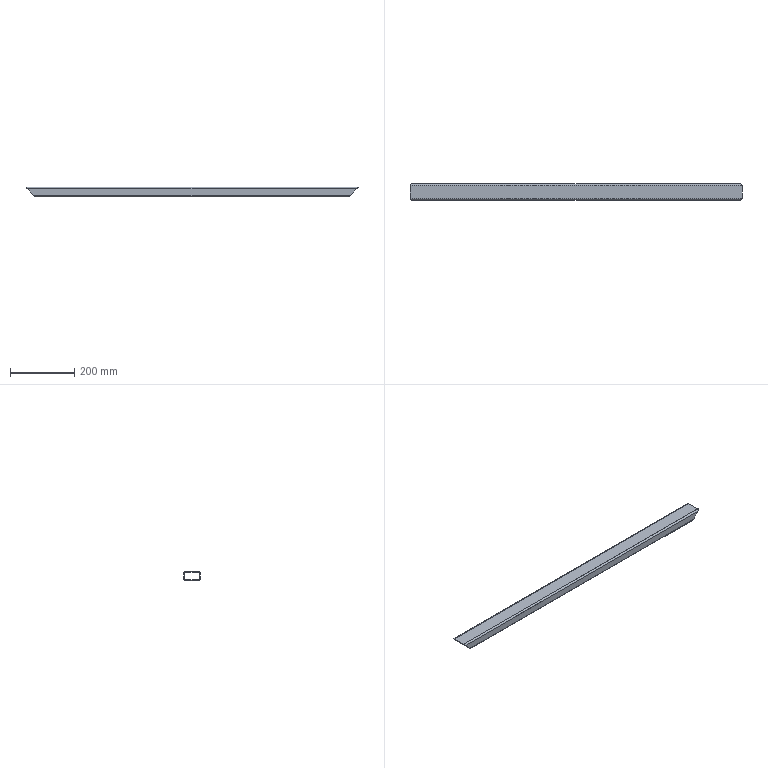Component | SolidWorks | Frame-1_SquareTube1-1 | 1 solid | 18 faces | box 1030 x 50 x 30 mm | volume 371551 mm3 | plane 10 | cylinder 8 | commonest cylinder face diameters 10.4 x4 5.2 x4
STEP:
#1=COLOUR_RGB('',0.7922,0.8196,0.9333);
#2=FILL_AREA_STYLE_COLOUR('',#1);
#3=FILL_AREA_STYLE('',(#2));
#4=SURFACE_STYLE_FILL_AREA(#3);
#5=SURFACE_SIDE_STYLE('',(#4));
#6=SURFACE_STYLE_USAGE(.BOTH.,#5);
#7=PRESENTATION_STYLE_ASSIGNMENT((#6));
#8=CARTESIAN_POINT('',(20.276,-0.7795,7.48));
#9=VERTEX_POINT('',#8);
#10=CARTESIAN_POINT('',(-20.276,-0.7795,7.48));
#11=VERTEX_POINT('',#10);
#12=CARTESIAN_POINT('',(19.685,-0.7795,7.48));
#13=DIRECTION('',(-1.,0.,0.));
#14=VECTOR('',#13,39.37);
#15=LINE('',#12,#14);
#16=EDGE_CURVE('',#9,#11,#15,.T.);
#17=ORIENTED_EDGE('',*,*,#16,.F.);
#18=CARTESIAN_POINT('',(20.276,0.7795,7.48));
#19=VERTEX_POINT('',#18);
#20=CARTESIAN_POINT('',(20.276,-0.7795,7.48));
#21=DIRECTION('',(0.,-1.,0.));
#22=VECTOR('',#21,39.37);
#23=LINE('',#20,#22);
#24=EDGE_CURVE('',#19,#9,#23,.T.);
#25=ORIENTED_EDGE('',*,*,#24,.F.);
#26=CARTESIAN_POINT('',(-20.276,0.7795,7.48));
#27=VERTEX_POINT('',#26);
#28=CARTESIAN_POINT('',(19.685,0.7795,7.48));
#29=DIRECTION('',(1.,0.,0.));
#30=VECTOR('',#29,39.37);
#31=LINE('',#28,#30);
#32=EDGE_CURVE('',#27,#19,#31,.T.);
#33=ORIENTED_EDGE('',*,*,#32,.F.);
#34=CARTESIAN_POINT('',(-20.276,-0.7795,7.48));
#35=DIRECTION('',(0.,1.,0.));
#36=VECTOR('',#35,39.37);
#37=LINE('',#34,#36);
#38=EDGE_CURVE('',#11,#27,#37,.T.);
#39=ORIENTED_EDGE('',*,*,#38,.F.);
#40=EDGE_LOOP('',(#17,#25,#33,#39));
#41=FACE_OUTER_BOUND('',#40,.T.);
#42=CARTESIAN_POINT('',(19.685,-0.7795,7.48));
#43=DIRECTION('',(0.,0.,-1.));
#44=DIRECTION('',(-1.,0.,0.));
#45=AXIS2_PLACEMENT_3D('',#42,#43,#44);
#46=PLANE('',#45);
#47=ADVANCED_FACE('',(#41),#46,.F.);
#48=ORIENTED_EDGE('',*,*,#38,.T.);
#49=CARTESIAN_POINT('',(-20.071,0.9843,7.276));
#50=VERTEX_POINT('',#49);
#51=CARTESIAN_POINT('',(-20.276,0.7795,7.48));
#52=CARTESIAN_POINT('',(-20.276,0.8995,7.48));
#53=CARTESIAN_POINT('',(-20.191,0.9843,7.396));
#54=CARTESIAN_POINT('',(-20.071,0.9843,7.276));
#55=(BOUNDED_CURVE()B_SPLINE_CURVE(3,(#51,#52,#53,#54),.UNSPECIFIED.,.F.,.F.)B_SPLINE_CURVE_WITH_KNOTS((4,4),(0.,1.571),.UNSPECIFIED.)CURVE()GEOMETRIC_REPRESENTATION_ITEM()RATIONAL_B_SPLINE_CURVE((1.,0.8047,0.8047,1.))REPRESENTATION_ITEM(''));
#56=EDGE_CURVE('',#27,#50,#55,.T.);
#57=ORIENTED_EDGE('',*,*,#56,.T.);
#58=CARTESIAN_POINT('',(-19.299,0.9843,6.504));
#59=VERTEX_POINT('',#58);
#60=CARTESIAN_POINT('',(-19.685,0.9843,6.89));
#61=DIRECTION('',(0.7071,0.,-0.7071));
#62=VECTOR('',#61,39.37);
#63=LINE('',#60,#62);
#64=EDGE_CURVE('',#50,#59,#63,.T.);
#65=ORIENTED_EDGE('',*,*,#64,.T.);
#66=CARTESIAN_POINT('',(-19.094,0.7795,6.299));
#67=VERTEX_POINT('',#66);
#68=CARTESIAN_POINT('',(-19.299,0.9843,6.504));
#69=CARTESIAN_POINT('',(-19.179,0.9843,6.384));
#70=CARTESIAN_POINT('',(-19.094,0.8995,6.299));
#71=CARTESIAN_POINT('',(-19.094,0.7795,6.299));
#72=(BOUNDED_CURVE()B_SPLINE_CURVE(3,(#68,#69,#70,#71),.UNSPECIFIED.,.F.,.T.)B_SPLINE_CURVE_WITH_KNOTS((4,4),(1.571,3.142),.UNSPECIFIED.)CURVE()GEOMETRIC_REPRESENTATION_ITEM()RATIONAL_B_SPLINE_CURVE((1.,0.8047,0.8047,1.))REPRESENTATION_ITEM(''));
#73=EDGE_CURVE('',#59,#67,#72,.T.);
#74=ORIENTED_EDGE('',*,*,#73,.T.);
#75=CARTESIAN_POINT('',(-19.094,-0.7795,6.299));
#76=VERTEX_POINT('',#75);
#77=CARTESIAN_POINT('',(-19.094,0.,6.299));
#78=DIRECTION('',(0.,-1.,0.));
#79=VECTOR('',#78,39.37);
#80=LINE('',#77,#79);
#81=EDGE_CURVE('',#67,#76,#80,.T.);
#82=ORIENTED_EDGE('',*,*,#81,.T.);
#83=CARTESIAN_POINT('',(-19.299,-0.9843,6.504));
#84=VERTEX_POINT('',#83);
#85=CARTESIAN_POINT('',(-19.094,-0.7795,6.299));
#86=CARTESIAN_POINT('',(-19.094,-0.8995,6.299));
#87=CARTESIAN_POINT('',(-19.179,-0.9843,6.384));
#88=CARTESIAN_POINT('',(-19.299,-0.9843,6.504));
#89=(BOUNDED_CURVE()B_SPLINE_CURVE(3,(#85,#86,#87,#88),.UNSPECIFIED.,.F.,.F.)B_SPLINE_CURVE_WITH_KNOTS((4,4),(3.142,4.712),.UNSPECIFIED.)CURVE()GEOMETRIC_REPRESENTATION_ITEM()RATIONAL_B_SPLINE_CURVE((1.,0.8047,0.8047,1.))REPRESENTATION_ITEM(''));
#90=EDGE_CURVE('',#76,#84,#89,.T.);
#91=ORIENTED_EDGE('',*,*,#90,.T.);
#92=CARTESIAN_POINT('',(-20.071,-0.9843,7.276));
#93=VERTEX_POINT('',#92);
#94=CARTESIAN_POINT('',(-19.685,-0.9843,6.89));
#95=DIRECTION('',(-0.7071,0.,0.7071));
#96=VECTOR('',#95,39.37);
#97=LINE('',#94,#96);
#98=EDGE_CURVE('',#84,#93,#97,.T.);
#99=ORIENTED_EDGE('',*,*,#98,.T.);
#100=CARTESIAN_POINT('',(-20.071,-0.9843,7.276));
#101=CARTESIAN_POINT('',(-20.191,-0.9843,7.396));
#102=CARTESIAN_POINT('',(-20.276,-0.8995,7.48));
#103=CARTESIAN_POINT('',(-20.276,-0.7795,7.48));
#104=(BOUNDED_CURVE()B_SPLINE_CURVE(3,(#100,#101,#102,#103),.UNSPECIFIED.,.F.,.F.)B_SPLINE_CURVE_WITH_KNOTS((4,4),(4.712,6.283),.UNSPECIFIED.)CURVE()GEOMETRIC_REPRESENTATION_ITEM()RATIONAL_B_SPLINE_CURVE((1.,0.8047,0.8047,1.))REPRESENTATION_ITEM(''));
#105=EDGE_CURVE('',#93,#11,#104,.T.);
#106=ORIENTED_EDGE('',*,*,#105,.T.);
#107=EDGE_LOOP('',(#48,#57,#65,#74,#82,#91,#99,#106));
#108=FACE_OUTER_BOUND('',#107,.T.);
#109=CARTESIAN_POINT('',(-19.197,0.7795,6.402));
#110=VERTEX_POINT('',#109);
#111=CARTESIAN_POINT('',(-19.299,0.8819,6.504));
#112=VERTEX_POINT('',#111);
#113=CARTESIAN_POINT('',(-19.197,0.7795,6.402));
#114=CARTESIAN_POINT('',(-19.197,0.8395,6.402));
#115=CARTESIAN_POINT('',(-19.239,0.8819,6.444));
#116=CARTESIAN_POINT('',(-19.299,0.8819,6.504));
#117=(BOUNDED_CURVE()B_SPLINE_CURVE(3,(#113,#114,#115,#116),.UNSPECIFIED.,.F.,.F.)B_SPLINE_CURVE_WITH_KNOTS((4,4),(3.142,4.712),.UNSPECIFIED.)CURVE()GEOMETRIC_REPRESENTATION_ITEM()RATIONAL_B_SPLINE_CURVE((1.,0.8047,0.8047,1.))REPRESENTATION_ITEM(''));
#118=EDGE_CURVE('',#110,#112,#117,.T.);
#119=ORIENTED_EDGE('',*,*,#118,.T.);
#120=CARTESIAN_POINT('',(-20.071,0.8819,7.276));
#121=VERTEX_POINT('',#120);
#122=CARTESIAN_POINT('',(-19.685,0.8819,6.89));
#123=DIRECTION('',(-0.7071,0.,0.7071));
#124=VECTOR('',#123,39.37);
#125=LINE('',#122,#124);
#126=EDGE_CURVE('',#112,#121,#125,.T.);
#127=ORIENTED_EDGE('',*,*,#126,.T.);
#128=CARTESIAN_POINT('',(-20.173,0.7795,7.378));
#129=VERTEX_POINT('',#128);
#130=CARTESIAN_POINT('',(-20.071,0.8819,7.276));
#131=CARTESIAN_POINT('',(-20.131,0.8819,7.336));
#132=CARTESIAN_POINT('',(-20.173,0.8395,7.378));
#133=CARTESIAN_POINT('',(-20.173,0.7795,7.378));
#134=(BOUNDED_CURVE()B_SPLINE_CURVE(3,(#130,#131,#132,#133),.UNSPECIFIED.,.F.,.T.)B_SPLINE_CURVE_WITH_KNOTS((4,4),(4.712,6.283),.UNSPECIFIED.)CURVE()GEOMETRIC_REPRESENTATION_ITEM()RATIONAL_B_SPLINE_CURVE((1.,0.8047,0.8047,1.))REPRESENTATION_ITEM(''));
#135=EDGE_CURVE('',#121,#129,#134,.T.);
#136=ORIENTED_EDGE('',*,*,#135,.T.);
#137=CARTESIAN_POINT('',(-20.173,-0.7795,7.378));
#138=VERTEX_POINT('',#137);
#139=CARTESIAN_POINT('',(-20.173,0.,7.378));
#140=DIRECTION('',(0.,-1.,0.));
#141=VECTOR('',#140,39.37);
#142=LINE('',#139,#141);
#143=EDGE_CURVE('',#129,#138,#142,.T.);
#144=ORIENTED_EDGE('',*,*,#143,.T.);
#145=CARTESIAN_POINT('',(-20.071,-0.8819,7.276));
#146=VERTEX_POINT('',#145);
#147=CARTESIAN_POINT('',(-20.173,-0.7795,7.378));
#148=CARTESIAN_POINT('',(-20.173,-0.8395,7.378));
#149=CARTESIAN_POINT('',(-20.131,-0.8819,7.336));
#150=CARTESIAN_POINT('',(-20.071,-0.8819,7.276));
#151=(BOUNDED_CURVE()B_SPLINE_CURVE(3,(#147,#148,#149,#150),.UNSPECIFIED.,.F.,.F.)B_SPLINE_CURVE_WITH_KNOTS((4,4),(0.,1.571),.UNSPECIFIED.)CURVE()GEOMETRIC_REPRESENTATION_ITEM()RATIONAL_B_SPLINE_CURVE((1.,0.8047,0.8047,1.))REPRESENTATION_ITEM(''));
#152=EDGE_CURVE('',#138,#146,#151,.T.);
#153=ORIENTED_EDGE('',*,*,#152,.T.);
#154=CARTESIAN_POINT('',(-19.299,-0.8819,6.504));
#155=VERTEX_POINT('',#154);
#156=CARTESIAN_POINT('',(-19.685,-0.8819,6.89));
#157=DIRECTION('',(0.7071,0.,-0.7071));
#158=VECTOR('',#157,39.37);
#159=LINE('',#156,#158);
#160=EDGE_CURVE('',#146,#155,#159,.T.);
#161=ORIENTED_EDGE('',*,*,#160,.T.);
#162=CARTESIAN_POINT('',(-19.197,-0.7795,6.402));
#163=VERTEX_POINT('',#162);
#164=CARTESIAN_POINT('',(-19.299,-0.8819,6.504));
#165=CARTESIAN_POINT('',(-19.239,-0.8819,6.444));
#166=CARTESIAN_POINT('',(-19.197,-0.8395,6.402));
#167=CARTESIAN_POINT('',(-19.197,-0.7795,6.402));
#168=(BOUNDED_CURVE()B_SPLINE_CURVE(3,(#164,#165,#166,#167),.UNSPECIFIED.,.F.,.F.)B_SPLINE_CURVE_WITH_KNOTS((4,4),(1.571,3.142),.UNSPECIFIED.)CURVE()GEOMETRIC_REPRESENTATION_ITEM()RATIONAL_B_SPLINE_CURVE((1.,0.8047,0.8047,1.))REPRESENTATION_ITEM(''));
#169=EDGE_CURVE('',#155,#163,#168,.T.);
#170=ORIENTED_EDGE('',*,*,#169,.T.);
#171=CARTESIAN_POINT('',(-19.197,0.,6.402));
#172=DIRECTION('',(0.,1.,0.));
#173=VECTOR('',#172,39.37);
#174=LINE('',#171,#173);
#175=EDGE_CURVE('',#163,#110,#174,.T.);
#176=ORIENTED_EDGE('',*,*,#175,.T.);
#177=EDGE_LOOP('',(#119,#127,#136,#144,#153,#161,#170,#176));
#178=FACE_BOUND('',#177,.T.);
#179=CARTESIAN_POINT('',(-19.685,0.,6.89));
#180=DIRECTION('',(-0.7071,0.,-0.7071));
#181=DIRECTION('',(-0.7071,0.,0.7071));
#182=AXIS2_PLACEMENT_3D('',#179,#180,#181);
#183=PLANE('',#182);
#184=ADVANCED_FACE('',(#108,#178),#183,.T.);
#185=CARTESIAN_POINT('',(20.071,-0.9843,7.276));
#186=VERTEX_POINT('',#185);
#187=CARTESIAN_POINT('',(20.071,-0.9843,7.276));
#188=CARTESIAN_POINT('',(20.191,-0.9843,7.396));
#189=CARTESIAN_POINT('',(20.276,-0.8995,7.48));
#190=CARTESIAN_POINT('',(20.276,-0.7795,7.48));
#191=(BOUNDED_CURVE()B_SPLINE_CURVE(3,(#187,#188,#189,#190),.UNSPECIFIED.,.F.,.F.)B_SPLINE_CURVE_WITH_KNOTS((4,4),(1.571,3.142),.UNSPECIFIED.)CURVE()GEOMETRIC_REPRESENTATION_ITEM()RATIONAL_B_SPLINE_CURVE((1.,0.8047,0.8047,1.))REPRESENTATION_ITEM(''));
#192=EDGE_CURVE('',#186,#9,#191,.T.);
#193=ORIENTED_EDGE('',*,*,#192,.T.);
#194=ORIENTED_EDGE('',*,*,#16,.T.);
#195=ORIENTED_EDGE('',*,*,#105,.F.);
#196=CARTESIAN_POINT('',(19.685,-0.9843,7.276));
#197=DIRECTION('',(1.,0.,0.));
#198=VECTOR('',#197,39.37);
#199=LINE('',#196,#198);
#200=EDGE_CURVE('',#93,#186,#199,.T.);
#201=ORIENTED_EDGE('',*,*,#200,.T.);
#202=EDGE_LOOP('',(#193,#194,#195,#201));
#203=FACE_OUTER_BOUND('',#202,.T.);
#204=CARTESIAN_POINT('',(19.685,-0.7795,7.276));
#205=DIRECTION('',(-1.,0.,0.));
#206=DIRECTION('',(0.,0.,1.));
#207=AXIS2_PLACEMENT_3D('',#204,#205,#206);
#208=CYLINDRICAL_SURFACE('',#207,0.2047);
#209=ADVANCED_FACE('',(#203),#208,.T.);
#210=CARTESIAN_POINT('',(19.299,-0.9843,6.504));
#211=VERTEX_POINT('',#210);
#212=CARTESIAN_POINT('',(19.685,-0.9843,6.89));
#213=DIRECTION('',(-0.7071,0.,-0.7071));
#214=VECTOR('',#213,39.37);
#215=LINE('',#212,#214);
#216=EDGE_CURVE('',#186,#211,#215,.T.);
#217=ORIENTED_EDGE('',*,*,#216,.T.);
#218=CARTESIAN_POINT('',(19.094,-0.7795,6.299));
#219=VERTEX_POINT('',#218);
#220=CARTESIAN_POINT('',(19.299,-0.9843,6.504));
#221=CARTESIAN_POINT('',(19.179,-0.9843,6.384));
#222=CARTESIAN_POINT('',(19.094,-0.8995,6.299));
#223=CARTESIAN_POINT('',(19.094,-0.7795,6.299));
#224=(BOUNDED_CURVE()B_SPLINE_CURVE(3,(#220,#221,#222,#223),.UNSPECIFIED.,.F.,.F.)B_SPLINE_CURVE_WITH_KNOTS((4,4),(4.712,6.283),.UNSPECIFIED.)CURVE()GEOMETRIC_REPRESENTATION_ITEM()RATIONAL_B_SPLINE_CURVE((1.,0.8047,0.8047,1.))REPRESENTATION_ITEM(''));
#225=EDGE_CURVE('',#211,#219,#224,.T.);
#226=ORIENTED_EDGE('',*,*,#225,.T.);
#227=CARTESIAN_POINT('',(19.094,0.7795,6.299));
#228=VERTEX_POINT('',#227);
#229=CARTESIAN_POINT('',(19.094,0.,6.299));
#230=DIRECTION('',(0.,1.,0.));
#231=VECTOR('',#230,39.37);
#232=LINE('',#229,#231);
#233=EDGE_CURVE('',#219,#228,#232,.T.);
#234=ORIENTED_EDGE('',*,*,#233,.T.);
#235=CARTESIAN_POINT('',(19.299,0.9843,6.504));
#236=VERTEX_POINT('',#235);
#237=CARTESIAN_POINT('',(19.094,0.7795,6.299));
#238=CARTESIAN_POINT('',(19.094,0.8995,6.299));
#239=CARTESIAN_POINT('',(19.179,0.9843,6.384));
#240=CARTESIAN_POINT('',(19.299,0.9843,6.504));
#241=(BOUNDED_CURVE()B_SPLINE_CURVE(3,(#237,#238,#239,#240),.UNSPECIFIED.,.F.,.F.)B_SPLINE_CURVE_WITH_KNOTS((4,4),(0.,1.571),.UNSPECIFIED.)CURVE()GEOMETRIC_REPRESENTATION_ITEM()RATIONAL_B_SPLINE_CURVE((1.,0.8047,0.8047,1.))REPRESENTATION_ITEM(''));
#242=EDGE_CURVE('',#228,#236,#241,.T.);
#243=ORIENTED_EDGE('',*,*,#242,.T.);
#244=CARTESIAN_POINT('',(20.071,0.9843,7.276));
#245=VERTEX_POINT('',#244);
#246=CARTESIAN_POINT('',(19.685,0.9843,6.89));
#247=DIRECTION('',(0.7071,0.,0.7071));
#248=VECTOR('',#247,39.37);
#249=LINE('',#246,#248);
#250=EDGE_CURVE('',#236,#245,#249,.T.);
#251=ORIENTED_EDGE('',*,*,#250,.T.);
#252=CARTESIAN_POINT('',(20.071,0.9843,7.276));
#253=CARTESIAN_POINT('',(20.191,0.9843,7.396));
#254=CARTESIAN_POINT('',(20.276,0.8995,7.48));
#255=CARTESIAN_POINT('',(20.276,0.7795,7.48));
#256=(BOUNDED_CURVE()B_SPLINE_CURVE(3,(#252,#253,#254,#255),.UNSPECIFIED.,.F.,.F.)B_SPLINE_CURVE_WITH_KNOTS((4,4),(1.571,3.142),.UNSPECIFIED.)CURVE()GEOMETRIC_REPRESENTATION_ITEM()RATIONAL_B_SPLINE_CURVE((1.,0.8047,0.8047,1.))REPRESENTATION_ITEM(''));
#257=EDGE_CURVE('',#245,#19,#256,.T.);
#258=ORIENTED_EDGE('',*,*,#257,.T.);
#259=ORIENTED_EDGE('',*,*,#24,.T.);
#260=ORIENTED_EDGE('',*,*,#192,.F.);
#261=EDGE_LOOP('',(#217,#226,#234,#243,#251,#258,#259,#260));
#262=FACE_OUTER_BOUND('',#261,.T.);
#263=CARTESIAN_POINT('',(20.071,-0.8819,7.276));
#264=VERTEX_POINT('',#263);
#265=CARTESIAN_POINT('',(20.173,-0.7795,7.378));
#266=VERTEX_POINT('',#265);
#267=CARTESIAN_POINT('',(20.071,-0.8819,7.276));
#268=CARTESIAN_POINT('',(20.131,-0.8819,7.336));
#269=CARTESIAN_POINT('',(20.173,-0.8395,7.378));
#270=CARTESIAN_POINT('',(20.173,-0.7795,7.378));
#271=(BOUNDED_CURVE()B_SPLINE_CURVE(3,(#267,#268,#269,#270),.UNSPECIFIED.,.F.,.F.)B_SPLINE_CURVE_WITH_KNOTS((4,4),(1.571,3.142),.UNSPECIFIED.)CURVE()GEOMETRIC_REPRESENTATION_ITEM()RATIONAL_B_SPLINE_CURVE((1.,0.8047,0.8047,1.))REPRESENTATION_ITEM(''));
#272=EDGE_CURVE('',#264,#266,#271,.T.);
#273=ORIENTED_EDGE('',*,*,#272,.T.);
#274=CARTESIAN_POINT('',(20.173,0.7795,7.378));
#275=VERTEX_POINT('',#274);
#276=CARTESIAN_POINT('',(20.173,0.,7.378));
#277=DIRECTION('',(0.,1.,0.));
#278=VECTOR('',#277,39.37);
#279=LINE('',#276,#278);
#280=EDGE_CURVE('',#266,#275,#279,.T.);
#281=ORIENTED_EDGE('',*,*,#280,.T.);
#282=CARTESIAN_POINT('',(20.071,0.8819,7.276));
#283=VERTEX_POINT('',#282);
#284=CARTESIAN_POINT('',(20.173,0.7795,7.378));
#285=CARTESIAN_POINT('',(20.173,0.8395,7.378));
#286=CARTESIAN_POINT('',(20.131,0.8819,7.336));
#287=CARTESIAN_POINT('',(20.071,0.8819,7.276));
#288=(BOUNDED_CURVE()B_SPLINE_CURVE(3,(#284,#285,#286,#287),.UNSPECIFIED.,.F.,.F.)B_SPLINE_CURVE_WITH_KNOTS((4,4),(3.142,4.712),.UNSPECIFIED.)CURVE()GEOMETRIC_REPRESENTATION_ITEM()RATIONAL_B_SPLINE_CURVE((1.,0.8047,0.8047,1.))REPRESENTATION_ITEM(''));
#289=EDGE_CURVE('',#275,#283,#288,.T.);
#290=ORIENTED_EDGE('',*,*,#289,.T.);
#291=CARTESIAN_POINT('',(19.299,0.8819,6.504));
#292=VERTEX_POINT('',#291);
#293=CARTESIAN_POINT('',(19.685,0.8819,6.89));
#294=DIRECTION('',(-0.7071,0.,-0.7071));
#295=VECTOR('',#294,39.37);
#296=LINE('',#293,#295);
#297=EDGE_CURVE('',#283,#292,#296,.T.);
#298=ORIENTED_EDGE('',*,*,#297,.T.);
#299=CARTESIAN_POINT('',(19.197,0.7795,6.402));
#300=VERTEX_POINT('',#299);
#301=CARTESIAN_POINT('',(19.299,0.8819,6.504));
#302=CARTESIAN_POINT('',(19.239,0.8819,6.444));
#303=CARTESIAN_POINT('',(19.197,0.8395,6.402));
#304=CARTESIAN_POINT('',(19.197,0.7795,6.402));
#305=(BOUNDED_CURVE()B_SPLINE_CURVE(3,(#301,#302,#303,#304),.UNSPECIFIED.,.F.,.F.)B_SPLINE_CURVE_WITH_KNOTS((4,4),(4.712,6.283),.UNSPECIFIED.)CURVE()GEOMETRIC_REPRESENTATION_ITEM()RATIONAL_B_SPLINE_CURVE((1.,0.8047,0.8047,1.))REPRESENTATION_ITEM(''));
#306=EDGE_CURVE('',#292,#300,#305,.T.);
#307=ORIENTED_EDGE('',*,*,#306,.T.);
#308=CARTESIAN_POINT('',(19.197,-0.7795,6.402));
#309=VERTEX_POINT('',#308);
#310=CARTESIAN_POINT('',(19.197,0.,6.402));
#311=DIRECTION('',(0.,-1.,0.));
#312=VECTOR('',#311,39.37);
#313=LINE('',#310,#312);
#314=EDGE_CURVE('',#300,#309,#313,.T.);
#315=ORIENTED_EDGE('',*,*,#314,.T.);
#316=CARTESIAN_POINT('',(19.299,-0.8819,6.504));
#317=VERTEX_POINT('',#316);
#318=CARTESIAN_POINT('',(19.197,-0.7795,6.402));
#319=CARTESIAN_POINT('',(19.197,-0.8395,6.402));
#320=CARTESIAN_POINT('',(19.239,-0.8819,6.444));
#321=CARTESIAN_POINT('',(19.299,-0.8819,6.504));
#322=(BOUNDED_CURVE()B_SPLINE_CURVE(3,(#318,#319,#320,#321),.UNSPECIFIED.,.F.,.T.)B_SPLINE_CURVE_WITH_KNOTS((4,4),(0.,1.571),.UNSPECIFIED.)CURVE()GEOMETRIC_REPRESENTATION_ITEM()RATIONAL_B_SPLINE_CURVE((1.,0.8047,0.8047,1.))REPRESENTATION_ITEM(''));
#323=EDGE_CURVE('',#309,#317,#322,.T.);
#324=ORIENTED_EDGE('',*,*,#323,.T.);
#325=CARTESIAN_POINT('',(19.685,-0.8819,6.89));
#326=DIRECTION('',(0.7071,0.,0.7071));
#327=VECTOR('',#326,39.37);
#328=LINE('',#325,#327);
#329=EDGE_CURVE('',#317,#264,#328,.T.);
#330=ORIENTED_EDGE('',*,*,#329,.T.);
#331=EDGE_LOOP('',(#273,#281,#290,#298,#307,#315,#324,#330));
#332=FACE_BOUND('',#331,.T.);
#333=CARTESIAN_POINT('',(19.685,0.,6.89));
#334=DIRECTION('',(0.7071,0.,-0.7071));
#335=DIRECTION('',(-0.7071,0.,-0.7071));
#336=AXIS2_PLACEMENT_3D('',#333,#334,#335);
#337=PLANE('',#336);
#338=ADVANCED_FACE('',(#262,#332),#337,.T.);
#339=ORIENTED_EDGE('',*,*,#257,.F.);
#340=CARTESIAN_POINT('',(19.685,0.9843,7.276));
#341=DIRECTION('',(-1.,0.,0.));
#342=VECTOR('',#341,39.37);
#343=LINE('',#340,#342);
#344=EDGE_CURVE('',#245,#50,#343,.T.);
#345=ORIENTED_EDGE('',*,*,#344,.T.);
#346=ORIENTED_EDGE('',*,*,#56,.F.);
#347=ORIENTED_EDGE('',*,*,#32,.T.);
#348=EDGE_LOOP('',(#339,#345,#346,#347));
#349=FACE_OUTER_BOUND('',#348,.T.);
#350=CARTESIAN_POINT('',(19.685,0.7795,7.276));
#351=DIRECTION('',(-1.,0.,0.));
#352=DIRECTION('',(0.,0.,1.));
#353=AXIS2_PLACEMENT_3D('',#350,#351,#352);
#354=CYLINDRICAL_SURFACE('',#353,0.2047);
#355=ADVANCED_FACE('',(#349),#354,.T.);
#356=CARTESIAN_POINT('',(19.685,-0.9843,6.504));
#357=DIRECTION('',(-1.,0.,0.));
#358=VECTOR('',#357,39.37);
#359=LINE('',#356,#358);
#360=EDGE_CURVE('',#211,#84,#359,.T.);
#361=ORIENTED_EDGE('',*,*,#360,.F.);
#362=ORIENTED_EDGE('',*,*,#216,.F.);
#363=ORIENTED_EDGE('',*,*,#200,.F.);
#364=ORIENTED_EDGE('',*,*,#98,.F.);
#365=EDGE_LOOP('',(#361,#362,#363,#364));
#366=FACE_OUTER_BOUND('',#365,.T.);
#367=CARTESIAN_POINT('',(19.685,-0.9843,7.276));
#368=DIRECTION('',(0.,1.,0.));
#369=DIRECTION('',(0.,0.,1.));
#370=AXIS2_PLACEMENT_3D('',#367,#368,#369);
#371=PLANE('',#370);
#372=ADVANCED_FACE('',(#366),#371,.F.);
#373=ORIENTED_EDGE('',*,*,#225,.F.);
#374=ORIENTED_EDGE('',*,*,#360,.T.);
#375=ORIENTED_EDGE('',*,*,#90,.F.);
#376=CARTESIAN_POINT('',(19.685,-0.7795,6.299));
#377=DIRECTION('',(1.,0.,0.));
#378=VECTOR('',#377,39.37);
#379=LINE('',#376,#378);
#380=EDGE_CURVE('',#76,#219,#379,.T.);
#381=ORIENTED_EDGE('',*,*,#380,.T.);
#382=EDGE_LOOP('',(#373,#374,#375,#381));
#383=FACE_OUTER_BOUND('',#382,.T.);
#384=CARTESIAN_POINT('',(19.685,-0.7795,6.504));
#385=DIRECTION('',(-1.,0.,0.));
#386=DIRECTION('',(0.,0.,1.));
#387=AXIS2_PLACEMENT_3D('',#384,#385,#386);
#388=CYLINDRICAL_SURFACE('',#387,0.2047);
#389=ADVANCED_FACE('',(#383),#388,.T.);
#390=CARTESIAN_POINT('',(19.685,0.7795,6.299));
#391=DIRECTION('',(-1.,0.,0.));
#392=VECTOR('',#391,39.37);
#393=LINE('',#390,#392);
#394=EDGE_CURVE('',#228,#67,#393,.T.);
#395=ORIENTED_EDGE('',*,*,#394,.F.);
#396=ORIENTED_EDGE('',*,*,#233,.F.);
#397=ORIENTED_EDGE('',*,*,#380,.F.);
#398=ORIENTED_EDGE('',*,*,#81,.F.);
#399=EDGE_LOOP('',(#395,#396,#397,#398));
#400=FACE_OUTER_BOUND('',#399,.T.);
#401=CARTESIAN_POINT('',(19.685,0.7795,6.299));
#402=DIRECTION('',(0.,0.,1.));
#403=DIRECTION('',(1.,0.,0.));
#404=AXIS2_PLACEMENT_3D('',#401,#402,#403);
#405=PLANE('',#404);
#406=ADVANCED_FACE('',(#400),#405,.F.);
#407=ORIENTED_EDGE('',*,*,#242,.F.);
#408=ORIENTED_EDGE('',*,*,#394,.T.);
#409=ORIENTED_EDGE('',*,*,#73,.F.);
#410=CARTESIAN_POINT('',(19.685,0.9843,6.504));
#411=DIRECTION('',(1.,0.,0.));
#412=VECTOR('',#411,39.37);
#413=LINE('',#410,#412);
#414=EDGE_CURVE('',#59,#236,#413,.T.);
#415=ORIENTED_EDGE('',*,*,#414,.T.);
#416=EDGE_LOOP('',(#407,#408,#409,#415));
#417=FACE_OUTER_BOUND('',#416,.T.);
#418=CARTESIAN_POINT('',(19.685,0.7795,6.504));
#419=DIRECTION('',(-1.,0.,0.));
#420=DIRECTION('',(0.,0.,1.));
#421=AXIS2_PLACEMENT_3D('',#418,#419,#420);
#422=CYLINDRICAL_SURFACE('',#421,0.2047);
#423=ADVANCED_FACE('',(#417),#422,.T.);
#424=ORIENTED_EDGE('',*,*,#344,.F.);
#425=ORIENTED_EDGE('',*,*,#250,.F.);
#426=ORIENTED_EDGE('',*,*,#414,.F.);
#427=ORIENTED_EDGE('',*,*,#64,.F.);
#428=EDGE_LOOP('',(#424,#425,#426,#427));
#429=FACE_OUTER_BOUND('',#428,.T.);
#430=CARTESIAN_POINT('',(19.685,0.9843,6.504));
#431=DIRECTION('',(0.,-1.,0.));
#432=DIRECTION('',(0.,0.,-1.));
#433=AXIS2_PLACEMENT_3D('',#430,#431,#432);
#434=PLANE('',#433);
#435=ADVANCED_FACE('',(#429),#434,.F.);
#436=CARTESIAN_POINT('',(19.685,0.8819,6.504));
#437=DIRECTION('',(1.,0.,0.));
#438=VECTOR('',#437,39.37);
#439=LINE('',#436,#438);
#440=EDGE_CURVE('',#112,#292,#439,.T.);
#441=ORIENTED_EDGE('',*,*,#440,.T.);
#442=ORIENTED_EDGE('',*,*,#297,.F.);
#443=CARTESIAN_POINT('',(19.685,0.8819,7.276));
#444=DIRECTION('',(-1.,0.,0.));
#445=VECTOR('',#444,39.37);
#446=LINE('',#443,#445);
#447=EDGE_CURVE('',#283,#121,#446,.T.);
#448=ORIENTED_EDGE('',*,*,#447,.T.);
#449=ORIENTED_EDGE('',*,*,#126,.F.);
#450=EDGE_LOOP('',(#441,#442,#448,#449));
#451=FACE_OUTER_BOUND('',#450,.T.);
#452=CARTESIAN_POINT('',(19.685,0.8819,6.504));
#453=DIRECTION('',(0.,-1.,0.));
#454=DIRECTION('',(0.,0.,-1.));
#455=AXIS2_PLACEMENT_3D('',#452,#453,#454);
#456=PLANE('',#455);
#457=ADVANCED_FACE('',(#451),#456,.T.);
#458=ORIENTED_EDGE('',*,*,#118,.F.);
#459=CARTESIAN_POINT('',(19.685,0.7795,6.402));
#460=DIRECTION('',(-1.,0.,0.));
#461=VECTOR('',#460,39.37);
#462=LINE('',#459,#461);
#463=EDGE_CURVE('',#300,#110,#462,.T.);
#464=ORIENTED_EDGE('',*,*,#463,.F.);
#465=ORIENTED_EDGE('',*,*,#306,.F.);
#466=ORIENTED_EDGE('',*,*,#440,.F.);
#467=EDGE_LOOP('',(#458,#464,#465,#466));
#468=FACE_OUTER_BOUND('',#467,.T.);
#469=CARTESIAN_POINT('',(19.685,0.7795,6.504));
#470=DIRECTION('',(-1.,0.,0.));
#471=DIRECTION('',(0.,0.,1.));
#472=AXIS2_PLACEMENT_3D('',#469,#470,#471);
#473=CYLINDRICAL_SURFACE('',#472,0.1024);
#474=ADVANCED_FACE('',(#468),#473,.F.);
#475=CARTESIAN_POINT('',(19.685,-0.7795,6.402));
#476=DIRECTION('',(1.,0.,0.));
#477=VECTOR('',#476,39.37);
#478=LINE('',#475,#477);
#479=EDGE_CURVE('',#163,#309,#478,.T.);
#480=ORIENTED_EDGE('',*,*,#479,.T.);
#481=ORIENTED_EDGE('',*,*,#314,.F.);
#482=ORIENTED_EDGE('',*,*,#463,.T.);
#483=ORIENTED_EDGE('',*,*,#175,.F.);
#484=EDGE_LOOP('',(#480,#481,#482,#483));
#485=FACE_OUTER_BOUND('',#484,.T.);
#486=CARTESIAN_POINT('',(19.685,0.7795,6.402));
#487=DIRECTION('',(0.,0.,1.));
#488=DIRECTION('',(1.,0.,0.));
#489=AXIS2_PLACEMENT_3D('',#486,#487,#488);
#490=PLANE('',#489);
#491=ADVANCED_FACE('',(#485),#490,.T.);
#492=ORIENTED_EDGE('',*,*,#169,.F.);
#493=CARTESIAN_POINT('',(19.685,-0.8819,6.504));
#494=DIRECTION('',(-1.,0.,0.));
#495=VECTOR('',#494,39.37);
#496=LINE('',#493,#495);
#497=EDGE_CURVE('',#317,#155,#496,.T.);
#498=ORIENTED_EDGE('',*,*,#497,.F.);
#499=ORIENTED_EDGE('',*,*,#323,.F.);
#500=ORIENTED_EDGE('',*,*,#479,.F.);
#501=EDGE_LOOP('',(#492,#498,#499,#500));
#502=FACE_OUTER_BOUND('',#501,.T.);
#503=CARTESIAN_POINT('',(19.685,-0.7795,6.504));
#504=DIRECTION('',(-1.,0.,0.));
#505=DIRECTION('',(0.,0.,1.));
#506=AXIS2_PLACEMENT_3D('',#503,#504,#505);
#507=CYLINDRICAL_SURFACE('',#506,0.1024);
#508=ADVANCED_FACE('',(#502),#507,.F.);
#509=CARTESIAN_POINT('',(19.685,-0.8819,7.276));
#510=DIRECTION('',(1.,0.,0.));
#511=VECTOR('',#510,39.37);
#512=LINE('',#509,#511);
#513=EDGE_CURVE('',#146,#264,#512,.T.);
#514=ORIENTED_EDGE('',*,*,#513,.T.);
#515=ORIENTED_EDGE('',*,*,#329,.F.);
#516=ORIENTED_EDGE('',*,*,#497,.T.);
#517=ORIENTED_EDGE('',*,*,#160,.F.);
#518=EDGE_LOOP('',(#514,#515,#516,#517));
#519=FACE_OUTER_BOUND('',#518,.T.);
#520=CARTESIAN_POINT('',(19.685,-0.8819,7.276));
#521=DIRECTION('',(0.,1.,0.));
#522=DIRECTION('',(0.,0.,1.));
#523=AXIS2_PLACEMENT_3D('',#520,#521,#522);
#524=PLANE('',#523);
#525=ADVANCED_FACE('',(#519),#524,.T.);
#526=ORIENTED_EDGE('',*,*,#152,.F.);
#527=CARTESIAN_POINT('',(19.685,-0.7795,7.378));
#528=DIRECTION('',(-1.,0.,0.));
#529=VECTOR('',#528,39.37);
#530=LINE('',#527,#529);
#531=EDGE_CURVE('',#266,#138,#530,.T.);
#532=ORIENTED_EDGE('',*,*,#531,.F.);
#533=ORIENTED_EDGE('',*,*,#272,.F.);
#534=ORIENTED_EDGE('',*,*,#513,.F.);
#535=EDGE_LOOP('',(#526,#532,#533,#534));
#536=FACE_OUTER_BOUND('',#535,.T.);
#537=CARTESIAN_POINT('',(19.685,-0.7795,7.276));
#538=DIRECTION('',(-1.,0.,0.));
#539=DIRECTION('',(0.,0.,1.));
#540=AXIS2_PLACEMENT_3D('',#537,#538,#539);
#541=CYLINDRICAL_SURFACE('',#540,0.1024);
#542=ADVANCED_FACE('',(#536),#541,.F.);
#543=CARTESIAN_POINT('',(19.685,0.7795,7.378));
#544=DIRECTION('',(1.,0.,0.));
#545=VECTOR('',#544,39.37);
#546=LINE('',#543,#545);
#547=EDGE_CURVE('',#129,#275,#546,.T.);
#548=ORIENTED_EDGE('',*,*,#547,.T.);
#549=ORIENTED_EDGE('',*,*,#280,.F.);
#550=ORIENTED_EDGE('',*,*,#531,.T.);
#551=ORIENTED_EDGE('',*,*,#143,.F.);
#552=EDGE_LOOP('',(#548,#549,#550,#551));
#553=FACE_OUTER_BOUND('',#552,.T.);
#554=CARTESIAN_POINT('',(19.685,-0.7795,7.378));
#555=DIRECTION('',(0.,0.,-1.));
#556=DIRECTION('',(-1.,0.,0.));
#557=AXIS2_PLACEMENT_3D('',#554,#555,#556);
#558=PLANE('',#557);
#559=ADVANCED_FACE('',(#553),#558,.T.);
#560=ORIENTED_EDGE('',*,*,#135,.F.);
#561=ORIENTED_EDGE('',*,*,#447,.F.);
#562=ORIENTED_EDGE('',*,*,#289,.F.);
#563=ORIENTED_EDGE('',*,*,#547,.F.);
#564=EDGE_LOOP('',(#560,#561,#562,#563));
#565=FACE_OUTER_BOUND('',#564,.T.);
#566=CARTESIAN_POINT('',(19.685,0.7795,7.276));
#567=DIRECTION('',(-1.,0.,0.));
#568=DIRECTION('',(0.,0.,1.));
#569=AXIS2_PLACEMENT_3D('',#566,#567,#568);
#570=CYLINDRICAL_SURFACE('',#569,0.1024);
#571=ADVANCED_FACE('',(#565),#570,.F.);
#572=CLOSED_SHELL('',(#47,#184,#209,#338,#355,#372,#389,#406,#423,#435,#457,#474,#491,#508,#525,#542,#559,#571));
#573=MANIFOLD_SOLID_BREP('',#572);
#574=STYLED_ITEM('',(#7),#573);
#575=PRESENTATION_LAYER_ASSIGNMENT('','',(#574));
#576=CARTESIAN_POINT('',(0.,0.,0.));
#577=DIRECTION('',(0.,0.,1.));
#578=DIRECTION('',(1.,0.,0.));
#579=AXIS2_PLACEMENT_3D('',#576,#577,#578);
#580=(LENGTH_UNIT()NAMED_UNIT(*)SI_UNIT($,.METRE.));
#581=LENGTH_MEASURE_WITH_UNIT(LENGTH_MEASURE(0.0254),#580);
#582=DIMENSIONAL_EXPONENTS(1.,0.,0.,0.,0.,0.,0.);
#583=(CONVERSION_BASED_UNIT('',#581)LENGTH_UNIT()NAMED_UNIT(#582));
#584=UNCERTAINTY_MEASURE_WITH_UNIT(LENGTH_MEASURE(0.00001),#583,'','');
#585=(NAMED_UNIT(*)PLANE_ANGLE_UNIT()SI_UNIT($,.RADIAN.));
#586=(NAMED_UNIT(*)SI_UNIT($,.STERADIAN.)SOLID_ANGLE_UNIT());
#587=(GEOMETRIC_REPRESENTATION_CONTEXT(3)GLOBAL_UNCERTAINTY_ASSIGNED_CONTEXT((#584))GLOBAL_UNIT_ASSIGNED_CONTEXT((#583,#585,#586))REPRESENTATION_CONTEXT('',''));
#588=ADVANCED_BREP_SHAPE_REPRESENTATION('',(#573,#579),#587);
#589=(LENGTH_UNIT()NAMED_UNIT(*)SI_UNIT($,.METRE.));
#590=LENGTH_MEASURE_WITH_UNIT(LENGTH_MEASURE(0.0254),#589);
#591=DIMENSIONAL_EXPONENTS(1.,0.,0.,0.,0.,0.,0.);
#592=(CONVERSION_BASED_UNIT('',#590)LENGTH_UNIT()NAMED_UNIT(#591));
#593=UNCERTAINTY_MEASURE_WITH_UNIT(LENGTH_MEASURE(0.00001),#592,'','');
#594=(NAMED_UNIT(*)PLANE_ANGLE_UNIT()SI_UNIT($,.RADIAN.));
#595=(NAMED_UNIT(*)SI_UNIT($,.STERADIAN.)SOLID_ANGLE_UNIT());
#596=(GEOMETRIC_REPRESENTATION_CONTEXT(3)GLOBAL_UNCERTAINTY_ASSIGNED_CONTEXT((#593))GLOBAL_UNIT_ASSIGNED_CONTEXT((#592,#594,#595))REPRESENTATION_CONTEXT('',''));
#597=MECHANICAL_DESIGN_GEOMETRIC_PRESENTATION_REPRESENTATION('',(#574),#596);